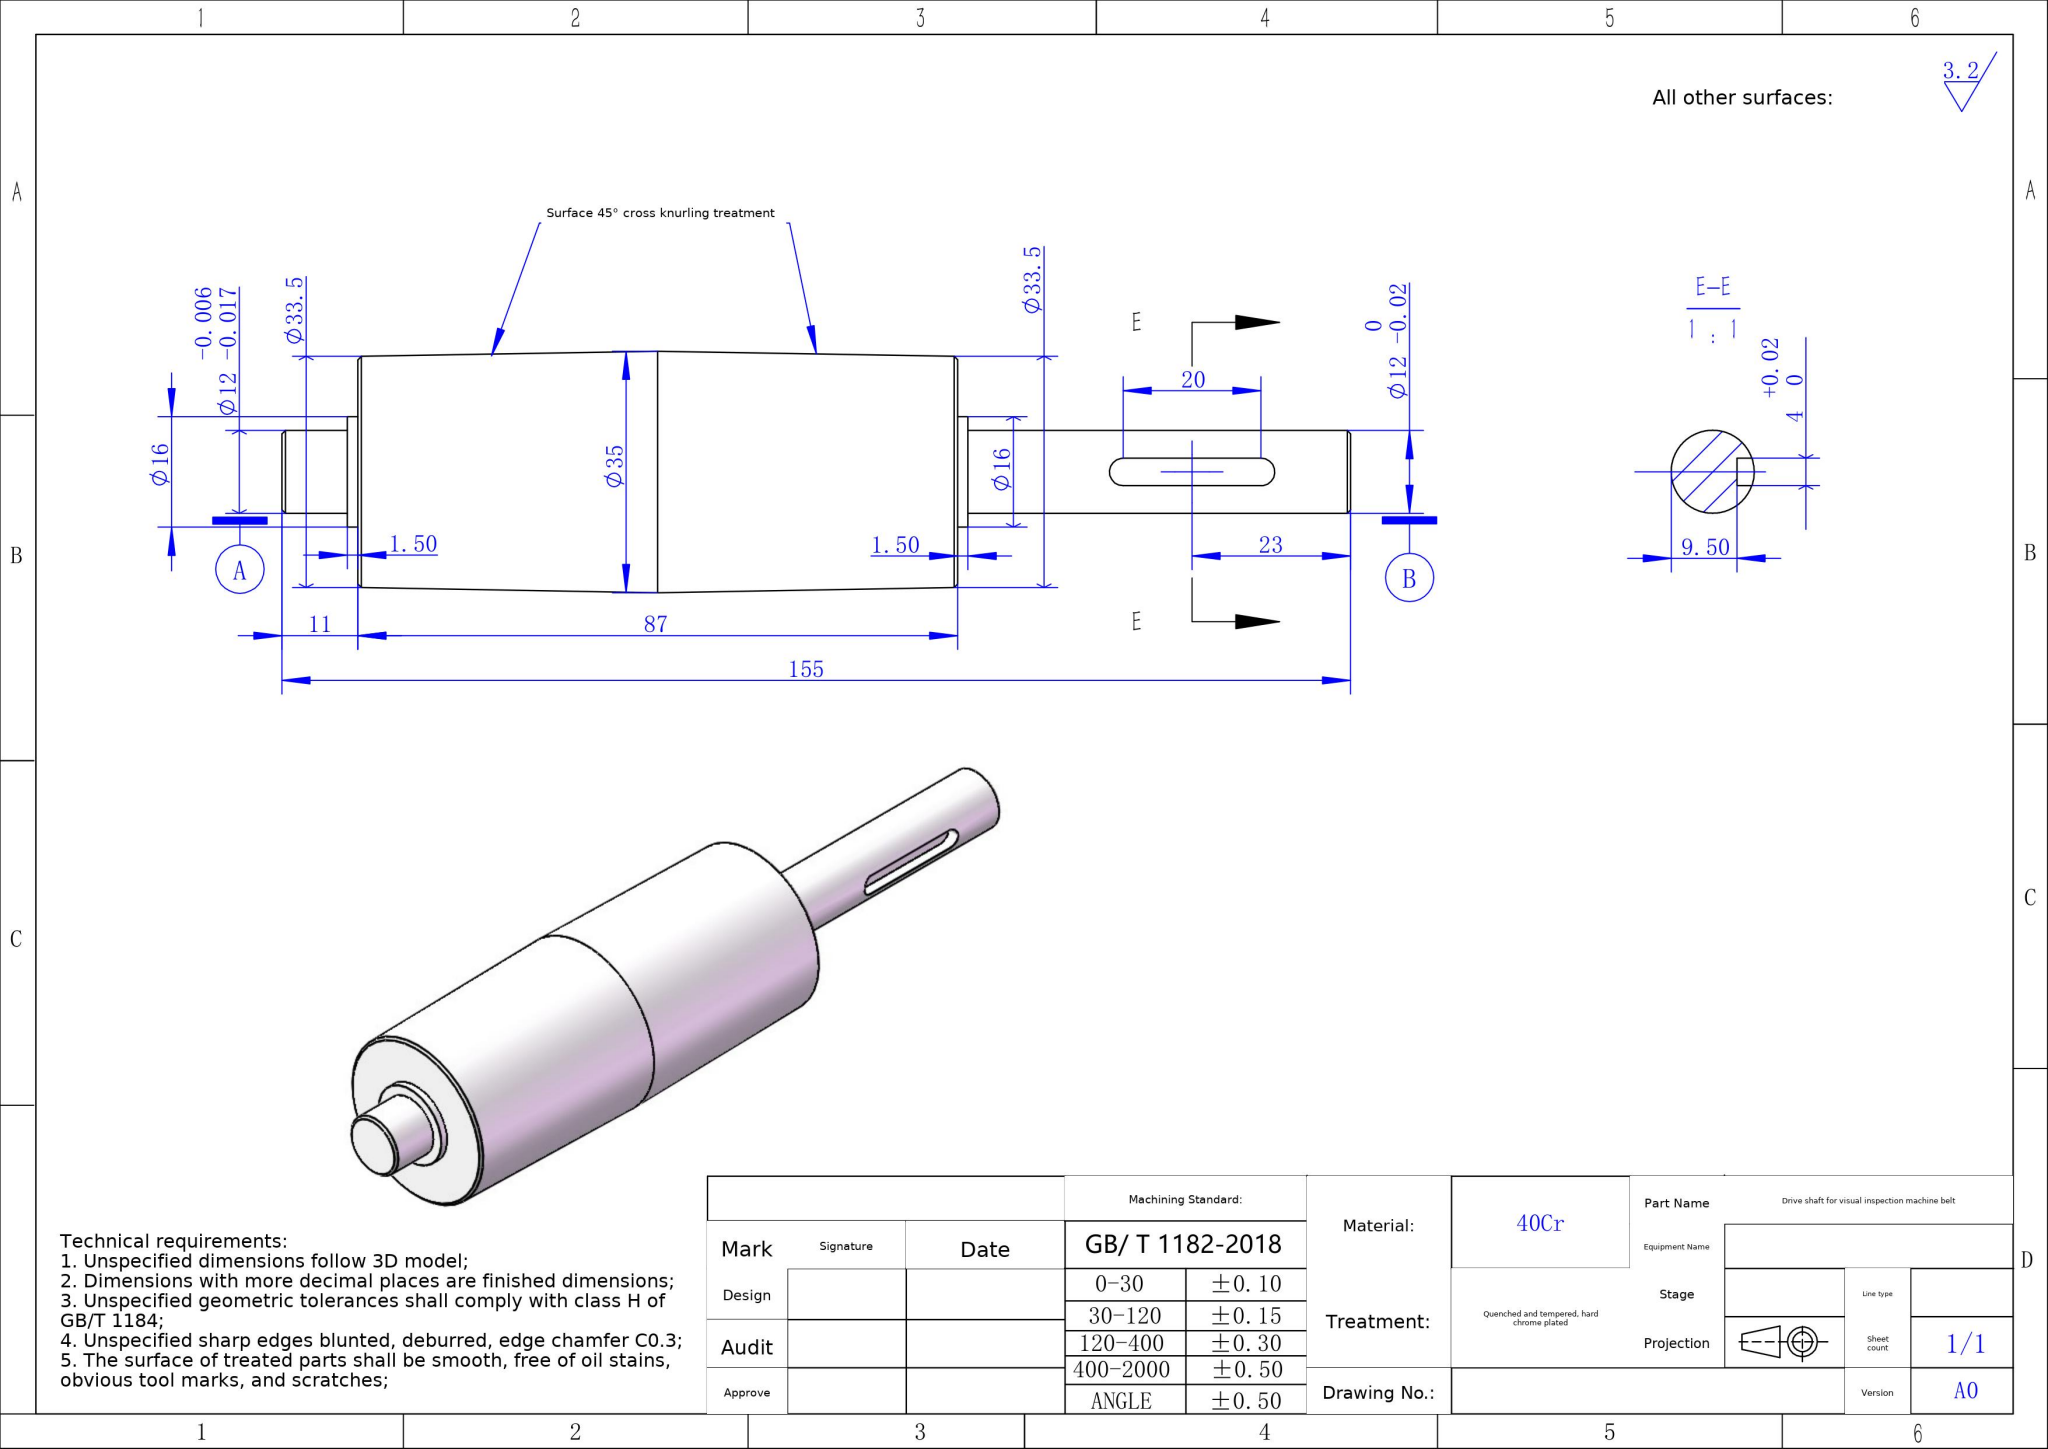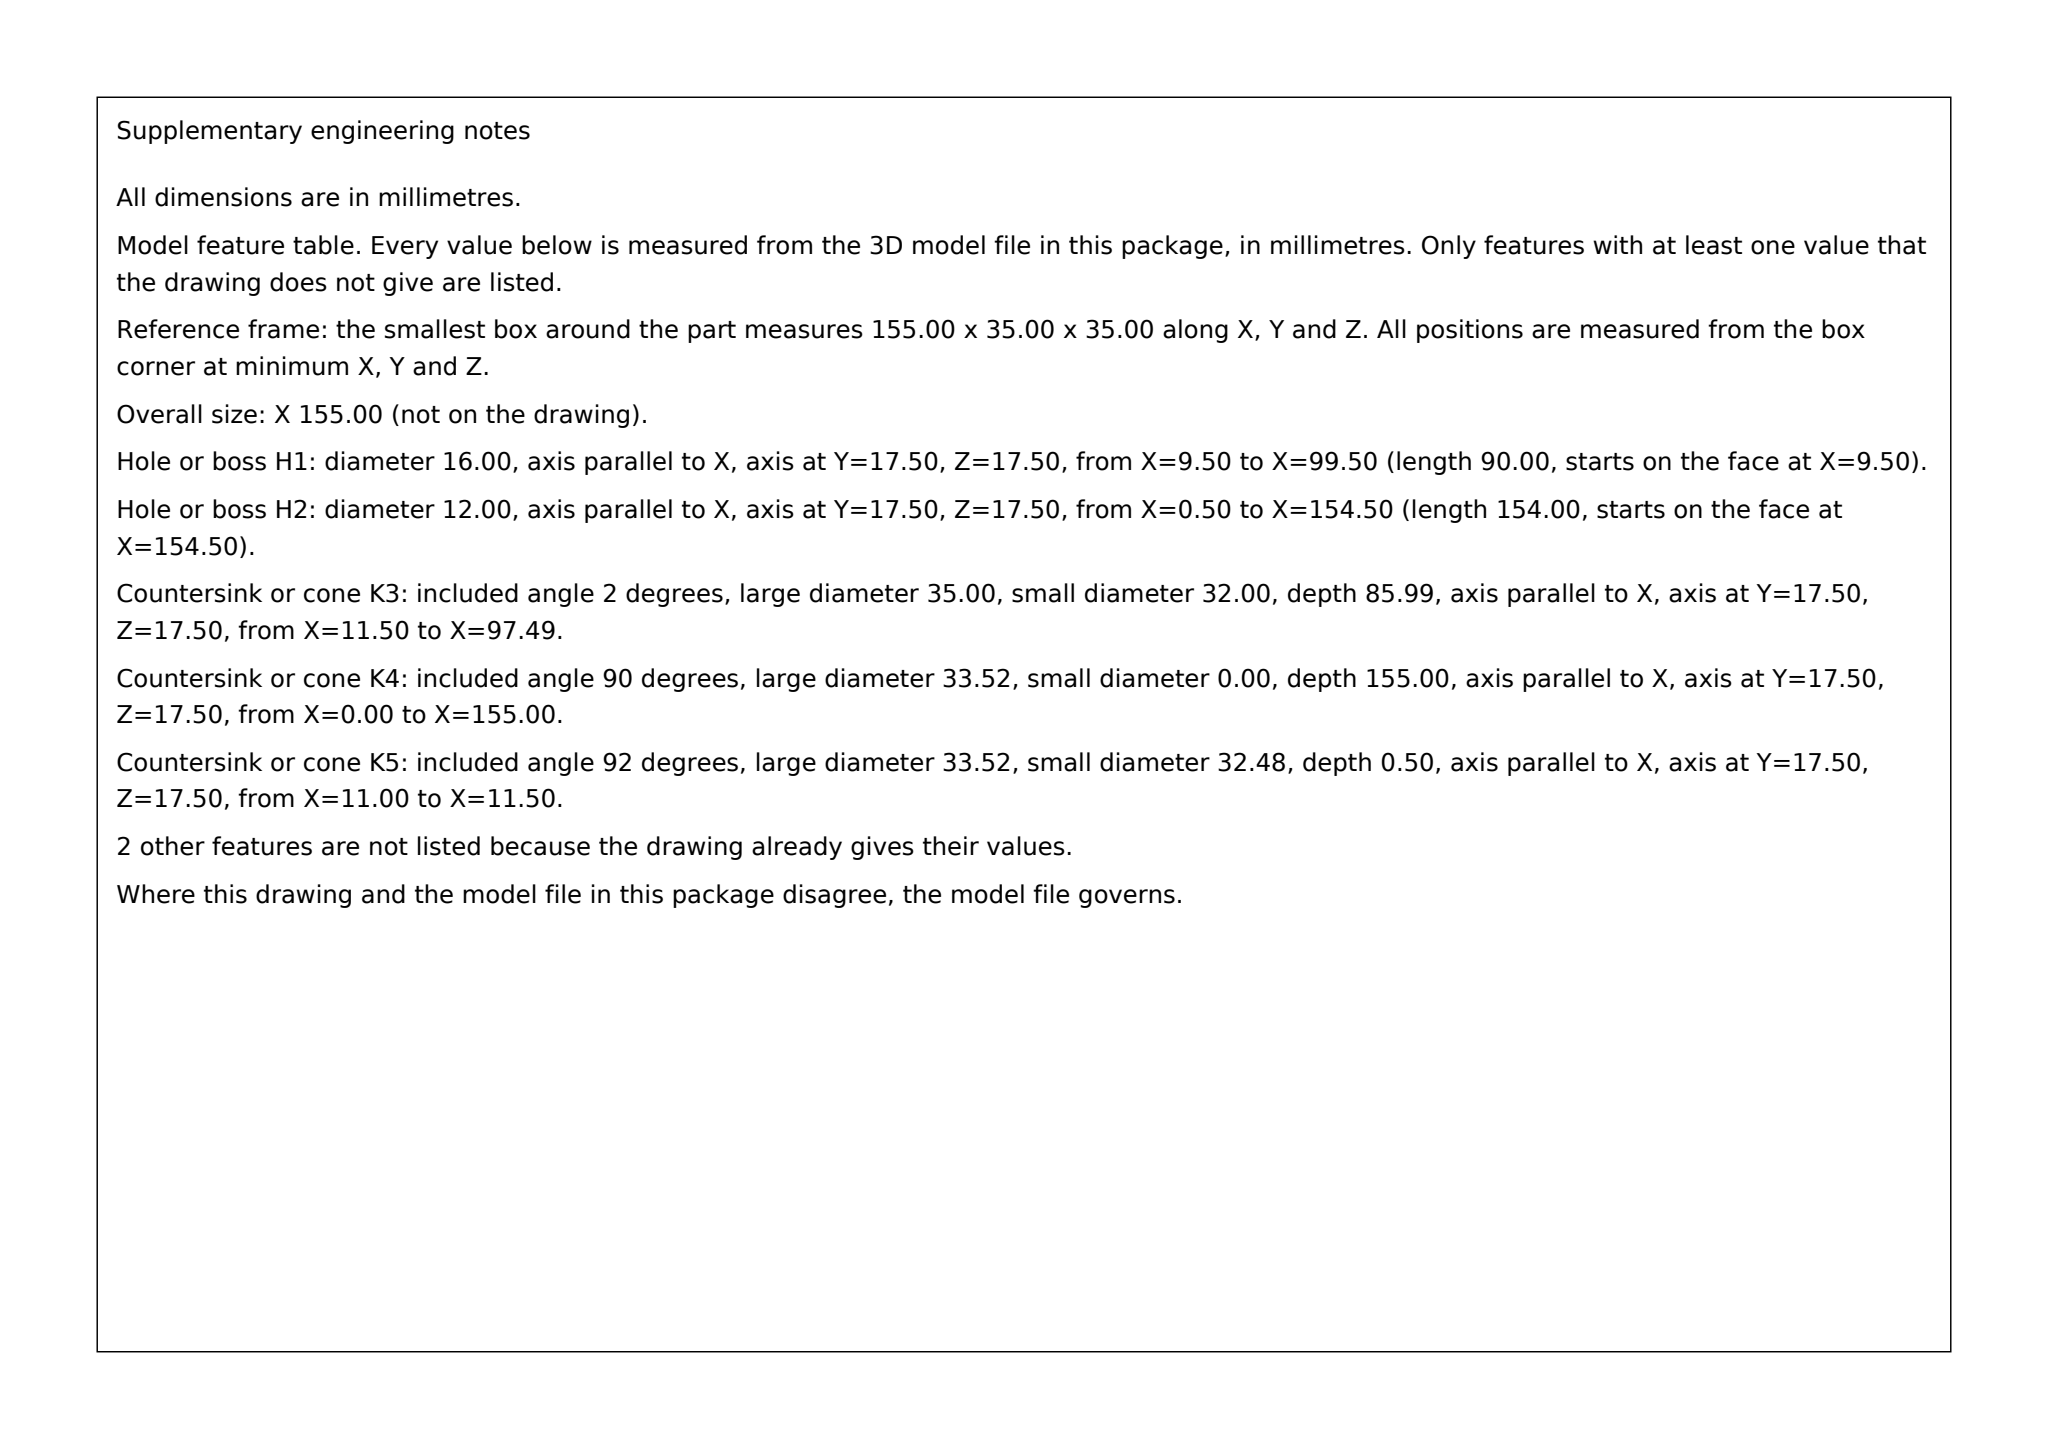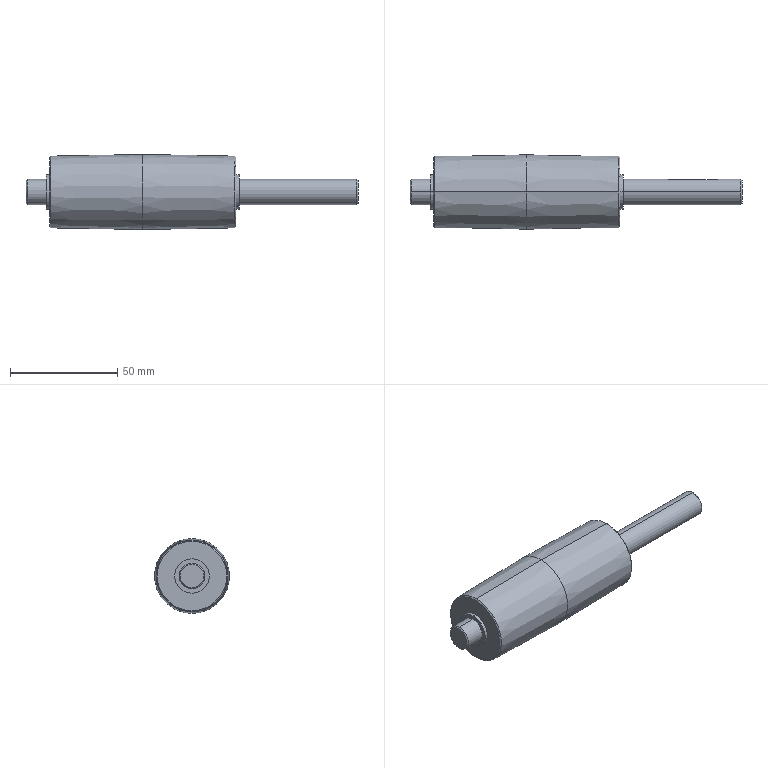Part | SolidWorks | mm | material 40Cr | 1 solid | 31 faces | box 155 x 35 x 35 mm | volume 87865 mm3 | cone 12 | cylinder 10 | plane 9 | commonest cylinder face diameters 12 x4 16 x4 4 x2
build123d program:
from build123d import *
from OCP.BRepFilletAPI import BRepFilletAPI_MakeChamfer

# Parameters (mm, degrees)
CUT_EXTRUDE1_DEPTH = 2.5
CHAMFER1_SIZE      = 0.5
CHAMFER1_SIZE2     = 0.5088


with BuildPart() as part:
    # Sketch1 → Revolve1 (revolve)
    with BuildSketch(Plane.XY, mode=Mode.PRIVATE) as revolve1_sk:
        Polygon((0, 0), (0, 6), (9.5, 6), (9.5, 8), (11, 8), (11, 16.75), (54.5, 17.5), (98, 16.75), (98, 8), (99.5, 8), (99.5, 6), (155, 6), (155, 0), align=None)
    revolve(revolve1_sk.sketch.rotate(Axis((0, 0, 0), (1, 0, 0)), 90), axis=Axis((0, 0, 0), (1, 0, 0)))

    # Sketch3 → Cut-Extrude1 (cut)
    with BuildSketch(Plane(origin=(155, 6, 0), x_dir=(1, 0, 0), z_dir=(0, 1, 0))):
        with BuildLine():
            Line((-33, 2), (-13, 2))
            ThreePointArc((-13, 2), (-11, 0), (-13, -2))
            Line((-13, -2), (-33, -2))
            ThreePointArc((-33, -2), (-35, 0), (-33, 2))
        make_face()
    extrude(amount=-CUT_EXTRUDE1_DEPTH, mode=Mode.SUBTRACT)

    # Chamfer1: one chamfer whose edges measure the first distance from different faces: ONE call of the kernel's chamfer builder (chamfer() names one face for all edges)
    chamfer1_edges_1 = [part.edges().sort_by_distance(p)[0] for p in [
        (155, 0, -6),
        (0, 0, -6),
    ]]
    chamfer1_edges_2 = [part.edges().sort_by_distance(p)[0] for p in [
        (98, 0, -16.75),
    ]]
    chamfer1_side_2 = [part.faces().sort_by_distance(p)[0] for p in [
        (98, 0, -16.276),
    ]]
    chamfer1_edges_3 = [part.edges().sort_by_distance(p)[0] for p in [
        (11, 0, -16.75),
    ]]
    chamfer1_side_3 = [part.faces().sort_by_distance(p)[0] for p in [
        (32.75, 0, -17.125),
    ]]
    chamfer1 = BRepFilletAPI_MakeChamfer(part.part.solid().wrapped)
    for e in chamfer1_edges_1:
        chamfer1.Add(CHAMFER1_SIZE, e.wrapped)
    for e in chamfer1_edges_2:
        chamfer1.Add(CHAMFER1_SIZE, CHAMFER1_SIZE2, e.wrapped, chamfer1_side_2[0].wrapped)  # the first distance lies on this face
    for e in chamfer1_edges_3:
        chamfer1.Add(CHAMFER1_SIZE, CHAMFER1_SIZE2, e.wrapped, chamfer1_side_3[0].wrapped)  # the first distance lies on this face
    add(Compound.cast(chamfer1.Shape()), mode=Mode.REPLACE)


solid = part.part
STEP:
#1=CARTESIAN_POINT('',(0.,0.,5.5));
#2=VERTEX_POINT('',#1);
#3=CARTESIAN_POINT('',(0.,0.,-5.5));
#4=VERTEX_POINT('',#3);
#5=CARTESIAN_POINT('',(0.,0.,0.));
#6=DIRECTION('',(-1.,0.,0.));
#7=DIRECTION('',(0.,0.,-1.));
#8=AXIS2_PLACEMENT_3D('',#5,#6,#7);
#9=CIRCLE('',#8,5.5);
#10=EDGE_CURVE('',#2,#4,#9,.T.);
#11=ORIENTED_EDGE('',*,*,#10,.F.);
#12=CARTESIAN_POINT('',(0.5,0.,6.));
#13=VERTEX_POINT('',#12);
#14=CARTESIAN_POINT('',(0.,0.,5.5));
#15=DIRECTION('',(0.7071,0.,0.7071));
#16=VECTOR('',#15,1000.);
#17=LINE('',#14,#16);
#18=EDGE_CURVE('',#2,#13,#17,.T.);
#19=ORIENTED_EDGE('',*,*,#18,.T.);
#20=CARTESIAN_POINT('',(0.5,0.,-6.));
#21=VERTEX_POINT('',#20);
#22=CARTESIAN_POINT('',(0.5,0.,0.));
#23=DIRECTION('',(1.,0.,0.));
#24=DIRECTION('',(0.,0.,-1.));
#25=AXIS2_PLACEMENT_3D('',#22,#23,#24);
#26=CIRCLE('',#25,6.);
#27=EDGE_CURVE('',#21,#13,#26,.T.);
#28=ORIENTED_EDGE('',*,*,#27,.F.);
#29=CARTESIAN_POINT('',(0.,0.,-5.5));
#30=DIRECTION('',(0.7071,0.,-0.7071));
#31=VECTOR('',#30,1000.);
#32=LINE('',#29,#31);
#33=EDGE_CURVE('',#4,#21,#32,.T.);
#34=ORIENTED_EDGE('',*,*,#33,.F.);
#35=EDGE_LOOP('',(#11,#19,#28,#34));
#36=FACE_OUTER_BOUND('',#35,.T.);
#37=CARTESIAN_POINT('',(0.,0.,0.));
#38=DIRECTION('',(1.,0.,0.));
#39=DIRECTION('',(0.,0.,-1.));
#40=AXIS2_PLACEMENT_3D('',#37,#38,#39);
#41=CONICAL_SURFACE('',#40,5.5,0.7854);
#42=ADVANCED_FACE('',(#36),#41,.T.);
#43=CARTESIAN_POINT('',(155.,0.,-5.5));
#44=VERTEX_POINT('',#43);
#45=CARTESIAN_POINT('',(155.,0.,5.5));
#46=VERTEX_POINT('',#45);
#47=CARTESIAN_POINT('',(155.,0.,0.));
#48=DIRECTION('',(1.,0.,0.));
#49=DIRECTION('',(0.,0.,1.));
#50=AXIS2_PLACEMENT_3D('',#47,#48,#49);
#51=CIRCLE('',#50,5.5);
#52=EDGE_CURVE('',#44,#46,#51,.T.);
#53=ORIENTED_EDGE('',*,*,#52,.F.);
#54=CARTESIAN_POINT('',(154.5,0.,-6.));
#55=VERTEX_POINT('',#54);
#56=CARTESIAN_POINT('',(154.5,0.,-6.));
#57=DIRECTION('',(-0.7071,0.,-0.7071));
#58=VECTOR('',#57,1000.);
#59=LINE('',#56,#58);
#60=EDGE_CURVE('',#44,#55,#59,.T.);
#61=ORIENTED_EDGE('',*,*,#60,.T.);
#62=CARTESIAN_POINT('',(154.5,0.,6.));
#63=VERTEX_POINT('',#62);
#64=CARTESIAN_POINT('',(154.5,0.,0.));
#65=DIRECTION('',(-1.,0.,0.));
#66=DIRECTION('',(0.,0.,1.));
#67=AXIS2_PLACEMENT_3D('',#64,#65,#66);
#68=CIRCLE('',#67,6.);
#69=EDGE_CURVE('',#63,#55,#68,.T.);
#70=ORIENTED_EDGE('',*,*,#69,.F.);
#71=CARTESIAN_POINT('',(154.5,0.,6.));
#72=DIRECTION('',(-0.7071,0.,0.7071));
#73=VECTOR('',#72,1000.);
#74=LINE('',#71,#73);
#75=EDGE_CURVE('',#46,#63,#74,.T.);
#76=ORIENTED_EDGE('',*,*,#75,.F.);
#77=EDGE_LOOP('',(#53,#61,#70,#76));
#78=FACE_OUTER_BOUND('',#77,.T.);
#79=CARTESIAN_POINT('',(154.5,0.,0.));
#80=DIRECTION('',(-1.,0.,0.));
#81=DIRECTION('',(0.,0.,1.));
#82=AXIS2_PLACEMENT_3D('',#79,#80,#81);
#83=CONICAL_SURFACE('',#82,6.,0.7854);
#84=ADVANCED_FACE('',(#78),#83,.T.);
#85=CARTESIAN_POINT('',(98.,0.,-16.25));
#86=VERTEX_POINT('',#85);
#87=CARTESIAN_POINT('',(98.,0.,16.25));
#88=VERTEX_POINT('',#87);
#89=CARTESIAN_POINT('',(98.,0.,0.));
#90=DIRECTION('',(1.,0.,0.));
#91=DIRECTION('',(0.,0.,1.));
#92=AXIS2_PLACEMENT_3D('',#89,#90,#91);
#93=CIRCLE('',#92,16.25);
#94=EDGE_CURVE('',#86,#88,#93,.T.);
#95=ORIENTED_EDGE('',*,*,#94,.F.);
#96=CARTESIAN_POINT('',(97.491,0.,-16.759));
#97=VERTEX_POINT('',#96);
#98=CARTESIAN_POINT('',(97.491,0.,-16.759));
#99=DIRECTION('',(-0.7071,0.,-0.7071));
#100=VECTOR('',#99,1000.);
#101=LINE('',#98,#100);
#102=EDGE_CURVE('',#86,#97,#101,.T.);
#103=ORIENTED_EDGE('',*,*,#102,.T.);
#104=CARTESIAN_POINT('',(97.491,0.,16.759));
#105=VERTEX_POINT('',#104);
#106=CARTESIAN_POINT('',(97.491,0.,0.));
#107=DIRECTION('',(-1.,0.,0.));
#108=DIRECTION('',(0.,0.,-1.));
#109=AXIS2_PLACEMENT_3D('',#106,#107,#108);
#110=CIRCLE('',#109,16.759);
#111=EDGE_CURVE('',#105,#97,#110,.T.);
#112=ORIENTED_EDGE('',*,*,#111,.F.);
#113=CARTESIAN_POINT('',(97.491,0.,16.759));
#114=DIRECTION('',(-0.7071,0.,0.7071));
#115=VECTOR('',#114,1000.);
#116=LINE('',#113,#115);
#117=EDGE_CURVE('',#88,#105,#116,.T.);
#118=ORIENTED_EDGE('',*,*,#117,.F.);
#119=EDGE_LOOP('',(#95,#103,#112,#118));
#120=FACE_OUTER_BOUND('',#119,.T.);
#121=CARTESIAN_POINT('',(97.491,0.,0.));
#122=DIRECTION('',(-1.,0.,0.));
#123=DIRECTION('',(0.,0.,1.));
#124=AXIS2_PLACEMENT_3D('',#121,#122,#123);
#125=CONICAL_SURFACE('',#124,16.759,0.7854);
#126=ADVANCED_FACE('',(#120),#125,.T.);
#127=CARTESIAN_POINT('',(11.,0.,16.241));
#128=VERTEX_POINT('',#127);
#129=CARTESIAN_POINT('',(11.,0.,-16.241));
#130=VERTEX_POINT('',#129);
#131=CARTESIAN_POINT('',(11.,0.,0.));
#132=DIRECTION('',(-1.,0.,0.));
#133=DIRECTION('',(0.,0.,-1.));
#134=AXIS2_PLACEMENT_3D('',#131,#132,#133);
#135=CIRCLE('',#134,16.241);
#136=EDGE_CURVE('',#128,#130,#135,.T.);
#137=ORIENTED_EDGE('',*,*,#136,.F.);
#138=CARTESIAN_POINT('',(11.5,0.,16.759));
#139=VERTEX_POINT('',#138);
#140=CARTESIAN_POINT('',(11.,0.,16.241));
#141=DIRECTION('',(0.6948,0.,0.7192));
#142=VECTOR('',#141,1000.);
#143=LINE('',#140,#142);
#144=EDGE_CURVE('',#128,#139,#143,.T.);
#145=ORIENTED_EDGE('',*,*,#144,.T.);
#146=CARTESIAN_POINT('',(11.5,0.,-16.759));
#147=VERTEX_POINT('',#146);
#148=CARTESIAN_POINT('',(11.5,0.,0.));
#149=DIRECTION('',(1.,0.,0.));
#150=DIRECTION('',(0.,0.,1.));
#151=AXIS2_PLACEMENT_3D('',#148,#149,#150);
#152=CIRCLE('',#151,16.759);
#153=EDGE_CURVE('',#147,#139,#152,.T.);
#154=ORIENTED_EDGE('',*,*,#153,.F.);
#155=CARTESIAN_POINT('',(11.,0.,-16.241));
#156=DIRECTION('',(0.6948,0.,-0.7192));
#157=VECTOR('',#156,1000.);
#158=LINE('',#155,#157);
#159=EDGE_CURVE('',#130,#147,#158,.T.);
#160=ORIENTED_EDGE('',*,*,#159,.F.);
#161=EDGE_LOOP('',(#137,#145,#154,#160));
#162=FACE_OUTER_BOUND('',#161,.T.);
#163=CARTESIAN_POINT('',(11.,0.,0.));
#164=DIRECTION('',(1.,0.,0.));
#165=DIRECTION('',(0.,0.,-1.));
#166=AXIS2_PLACEMENT_3D('',#163,#164,#165);
#167=CONICAL_SURFACE('',#166,16.241,0.8026);
#168=ADVANCED_FACE('',(#162),#167,.T.);
#169=CARTESIAN_POINT('',(122.,5.657,-2.));
#170=VERTEX_POINT('',#169);
#171=CARTESIAN_POINT('',(142.,5.657,-2.));
#172=VERTEX_POINT('',#171);
#173=CARTESIAN_POINT('',(0.,5.657,-2.));
#174=DIRECTION('',(1.,0.,0.));
#175=VECTOR('',#174,1000.);
#176=LINE('',#173,#175);
#177=EDGE_CURVE('',#170,#172,#176,.T.);
#178=ORIENTED_EDGE('',*,*,#177,.T.);
#179=CARTESIAN_POINT('',(142.,5.657,2.));
#180=VERTEX_POINT('',#179);
#181=CARTESIAN_POINT('',(142.,5.657,-2.));
#182=CARTESIAN_POINT('',(142.133,5.657,-2.));
#183=CARTESIAN_POINT('',(142.264,5.662,-1.987));
#184=CARTESIAN_POINT('',(142.521,5.679,-1.935));
#185=CARTESIAN_POINT('',(142.648,5.693,-1.897));
#186=CARTESIAN_POINT('',(142.89,5.725,-1.796));
#187=CARTESIAN_POINT('',(143.004,5.744,-1.735));
#188=CARTESIAN_POINT('',(143.221,5.786,-1.59));
#189=CARTESIAN_POINT('',(143.323,5.809,-1.506));
#190=CARTESIAN_POINT('',(143.597,5.875,-1.231));
#191=CARTESIAN_POINT('',(143.746,5.919,-1.01));
#192=CARTESIAN_POINT('',(143.896,5.966,-0.6496));
#193=CARTESIAN_POINT('',(143.935,5.979,-0.5226));
#194=CARTESIAN_POINT('',(143.987,5.996,-0.264));
#195=CARTESIAN_POINT('',(144.,6.,-0.1336));
#196=CARTESIAN_POINT('',(144.,6.,0.1294));
#197=CARTESIAN_POINT('',(143.987,5.996,0.2629));
#198=CARTESIAN_POINT('',(143.936,5.979,0.5202));
#199=CARTESIAN_POINT('',(143.898,5.966,0.6454));
#200=CARTESIAN_POINT('',(143.796,5.935,0.8889));
#201=CARTESIAN_POINT('',(143.734,5.916,1.004));
#202=CARTESIAN_POINT('',(143.59,5.876,1.22));
#203=CARTESIAN_POINT('',(143.507,5.853,1.322));
#204=CARTESIAN_POINT('',(143.323,5.809,1.506));
#205=CARTESIAN_POINT('',(143.223,5.787,1.588));
#206=CARTESIAN_POINT('',(143.007,5.745,1.733));
#207=CARTESIAN_POINT('',(142.89,5.725,1.796));
#208=CARTESIAN_POINT('',(142.529,5.677,1.946));
#209=CARTESIAN_POINT('',(142.266,5.657,2.));
#210=CARTESIAN_POINT('',(142.,5.657,2.));
#211=B_SPLINE_CURVE_WITH_KNOTS('',3,(#181,#182,#183,#184,#185,#186,#187,#188,#189,#190,#191,#192,#193,#194,#195,#196,#197,#198,#199,#200,#201,#202,#203,#204,#205,#206,#207,#208,#209,#210),.UNSPECIFIED.,.F.,.F.,(4,2,2,2,2,2,2,2,2,2,2,2,2,2,4),(0.,0.0003935,0.000787,0.00118,0.001574,0.002361,0.002754,0.003148,0.003541,0.003935,0.004328,0.004722,0.005115,0.005509,0.006296),.UNSPECIFIED.);
#212=EDGE_CURVE('',#172,#180,#211,.T.);
#213=ORIENTED_EDGE('',*,*,#212,.T.);
#214=CARTESIAN_POINT('',(122.,5.657,2.));
#215=VERTEX_POINT('',#214);
#216=CARTESIAN_POINT('',(0.,5.657,2.));
#217=DIRECTION('',(-1.,0.,0.));
#218=VECTOR('',#217,1000.);
#219=LINE('',#216,#218);
#220=EDGE_CURVE('',#180,#215,#219,.T.);
#221=ORIENTED_EDGE('',*,*,#220,.T.);
#222=CARTESIAN_POINT('',(122.,5.657,2.));
#223=CARTESIAN_POINT('',(121.867,5.657,2.));
#224=CARTESIAN_POINT('',(121.736,5.662,1.987));
#225=CARTESIAN_POINT('',(121.479,5.679,1.935));
#226=CARTESIAN_POINT('',(121.352,5.693,1.897));
#227=CARTESIAN_POINT('',(121.11,5.725,1.796));
#228=CARTESIAN_POINT('',(120.996,5.744,1.735));
#229=CARTESIAN_POINT('',(120.779,5.786,1.59));
#230=CARTESIAN_POINT('',(120.677,5.809,1.506));
#231=CARTESIAN_POINT('',(120.403,5.875,1.231));
#232=CARTESIAN_POINT('',(120.254,5.919,1.01));
#233=CARTESIAN_POINT('',(120.104,5.966,0.6496));
#234=CARTESIAN_POINT('',(120.065,5.979,0.5226));
#235=CARTESIAN_POINT('',(120.013,5.996,0.264));
#236=CARTESIAN_POINT('',(120.,6.,0.1336));
#237=CARTESIAN_POINT('',(120.,6.,-0.1294));
#238=CARTESIAN_POINT('',(120.013,5.996,-0.2629));
#239=CARTESIAN_POINT('',(120.064,5.979,-0.5202));
#240=CARTESIAN_POINT('',(120.102,5.966,-0.6454));
#241=CARTESIAN_POINT('',(120.204,5.935,-0.8889));
#242=CARTESIAN_POINT('',(120.266,5.916,-1.004));
#243=CARTESIAN_POINT('',(120.41,5.876,-1.22));
#244=CARTESIAN_POINT('',(120.493,5.853,-1.322));
#245=CARTESIAN_POINT('',(120.677,5.809,-1.506));
#246=CARTESIAN_POINT('',(120.777,5.787,-1.588));
#247=CARTESIAN_POINT('',(120.993,5.745,-1.733));
#248=CARTESIAN_POINT('',(121.11,5.725,-1.796));
#249=CARTESIAN_POINT('',(121.471,5.677,-1.946));
#250=CARTESIAN_POINT('',(121.734,5.657,-2.));
#251=CARTESIAN_POINT('',(122.,5.657,-2.));
#252=B_SPLINE_CURVE_WITH_KNOTS('',3,(#222,#223,#224,#225,#226,#227,#228,#229,#230,#231,#232,#233,#234,#235,#236,#237,#238,#239,#240,#241,#242,#243,#244,#245,#246,#247,#248,#249,#250,#251),.UNSPECIFIED.,.F.,.F.,(4,2,2,2,2,2,2,2,2,2,2,2,2,2,4),(0.,0.0003935,0.000787,0.00118,0.001574,0.002361,0.002754,0.003148,0.003541,0.003935,0.004328,0.004722,0.005115,0.005509,0.006296),.UNSPECIFIED.);
#253=EDGE_CURVE('',#215,#170,#252,.T.);
#254=ORIENTED_EDGE('',*,*,#253,.T.);
#255=EDGE_LOOP('',(#178,#213,#221,#254));
#256=FACE_BOUND('',#255,.T.);
#257=ORIENTED_EDGE('',*,*,#69,.T.);
#258=CARTESIAN_POINT('',(99.5,0.,-6.));
#259=VERTEX_POINT('',#258);
#260=CARTESIAN_POINT('',(0.,0.,-6.));
#261=DIRECTION('',(-1.,0.,0.));
#262=VECTOR('',#261,1000.);
#263=LINE('',#260,#262);
#264=EDGE_CURVE('',#55,#259,#263,.T.);
#265=ORIENTED_EDGE('',*,*,#264,.T.);
#266=CARTESIAN_POINT('',(99.5,0.,6.));
#267=VERTEX_POINT('',#266);
#268=CARTESIAN_POINT('',(99.5,0.,0.));
#269=DIRECTION('',(-1.,0.,0.));
#270=DIRECTION('',(0.,0.,1.));
#271=AXIS2_PLACEMENT_3D('',#268,#269,#270);
#272=CIRCLE('',#271,6.);
#273=EDGE_CURVE('',#267,#259,#272,.T.);
#274=ORIENTED_EDGE('',*,*,#273,.F.);
#275=CARTESIAN_POINT('',(0.,0.,6.));
#276=DIRECTION('',(-1.,0.,0.));
#277=VECTOR('',#276,1000.);
#278=LINE('',#275,#277);
#279=EDGE_CURVE('',#63,#267,#278,.T.);
#280=ORIENTED_EDGE('',*,*,#279,.F.);
#281=EDGE_LOOP('',(#257,#265,#274,#280));
#282=FACE_OUTER_BOUND('',#281,.T.);
#283=CARTESIAN_POINT('',(0.,0.,0.));
#284=DIRECTION('',(-1.,0.,0.));
#285=DIRECTION('',(0.,0.,1.));
#286=AXIS2_PLACEMENT_3D('',#283,#284,#285);
#287=CYLINDRICAL_SURFACE('',#286,6.);
#288=ADVANCED_FACE('',(#256,#282),#287,.T.);
#289=CARTESIAN_POINT('',(99.5,0.,8.));
#290=VERTEX_POINT('',#289);
#291=CARTESIAN_POINT('',(99.5,0.,-8.));
#292=VERTEX_POINT('',#291);
#293=CARTESIAN_POINT('',(99.5,0.,0.));
#294=DIRECTION('',(-1.,0.,0.));
#295=DIRECTION('',(0.,0.,1.));
#296=AXIS2_PLACEMENT_3D('',#293,#294,#295);
#297=CIRCLE('',#296,8.);
#298=EDGE_CURVE('',#290,#292,#297,.T.);
#299=ORIENTED_EDGE('',*,*,#298,.T.);
#300=CARTESIAN_POINT('',(98.,0.,-8.));
#301=VERTEX_POINT('',#300);
#302=CARTESIAN_POINT('',(0.,0.,-8.));
#303=DIRECTION('',(-1.,0.,0.));
#304=VECTOR('',#303,1000.);
#305=LINE('',#302,#304);
#306=EDGE_CURVE('',#292,#301,#305,.T.);
#307=ORIENTED_EDGE('',*,*,#306,.T.);
#308=CARTESIAN_POINT('',(98.,0.,8.));
#309=VERTEX_POINT('',#308);
#310=CARTESIAN_POINT('',(98.,0.,0.));
#311=DIRECTION('',(-1.,0.,0.));
#312=DIRECTION('',(0.,0.,1.));
#313=AXIS2_PLACEMENT_3D('',#310,#311,#312);
#314=CIRCLE('',#313,8.);
#315=EDGE_CURVE('',#309,#301,#314,.T.);
#316=ORIENTED_EDGE('',*,*,#315,.F.);
#317=CARTESIAN_POINT('',(0.,0.,8.));
#318=DIRECTION('',(-1.,0.,0.));
#319=VECTOR('',#318,1000.);
#320=LINE('',#317,#319);
#321=EDGE_CURVE('',#290,#309,#320,.T.);
#322=ORIENTED_EDGE('',*,*,#321,.F.);
#323=EDGE_LOOP('',(#299,#307,#316,#322));
#324=FACE_OUTER_BOUND('',#323,.T.);
#325=CARTESIAN_POINT('',(0.,0.,0.));
#326=DIRECTION('',(-1.,0.,0.));
#327=DIRECTION('',(0.,0.,1.));
#328=AXIS2_PLACEMENT_3D('',#325,#326,#327);
#329=CYLINDRICAL_SURFACE('',#328,8.);
#330=ADVANCED_FACE('',(#324),#329,.T.);
#331=ORIENTED_EDGE('',*,*,#111,.T.);
#332=CARTESIAN_POINT('',(54.5,0.,-17.5));
#333=VERTEX_POINT('',#332);
#334=CARTESIAN_POINT('',(98.,0.,-16.75));
#335=DIRECTION('',(-0.9999,0.,-0.01724));
#336=VECTOR('',#335,1000.);
#337=LINE('',#334,#336);
#338=EDGE_CURVE('',#97,#333,#337,.T.);
#339=ORIENTED_EDGE('',*,*,#338,.T.);
#340=CARTESIAN_POINT('',(54.5,0.,17.5));
#341=VERTEX_POINT('',#340);
#342=CARTESIAN_POINT('',(54.5,0.,0.));
#343=DIRECTION('',(-1.,0.,0.));
#344=DIRECTION('',(0.,0.,1.));
#345=AXIS2_PLACEMENT_3D('',#342,#343,#344);
#346=CIRCLE('',#345,17.5);
#347=EDGE_CURVE('',#341,#333,#346,.T.);
#348=ORIENTED_EDGE('',*,*,#347,.F.);
#349=CARTESIAN_POINT('',(98.,0.,16.75));
#350=DIRECTION('',(-0.9999,0.,0.01724));
#351=VECTOR('',#350,1000.);
#352=LINE('',#349,#351);
#353=EDGE_CURVE('',#105,#341,#352,.T.);
#354=ORIENTED_EDGE('',*,*,#353,.F.);
#355=EDGE_LOOP('',(#331,#339,#348,#354));
#356=FACE_OUTER_BOUND('',#355,.T.);
#357=CARTESIAN_POINT('',(98.,0.,0.));
#358=DIRECTION('',(-1.,0.,0.));
#359=DIRECTION('',(0.,0.,1.));
#360=AXIS2_PLACEMENT_3D('',#357,#358,#359);
#361=CONICAL_SURFACE('',#360,16.75,0.01724);
#362=ADVANCED_FACE('',(#356),#361,.T.);
#363=ORIENTED_EDGE('',*,*,#153,.T.);
#364=CARTESIAN_POINT('',(54.5,0.,17.5));
#365=DIRECTION('',(0.9999,0.,0.01724));
#366=VECTOR('',#365,1000.);
#367=LINE('',#364,#366);
#368=EDGE_CURVE('',#139,#341,#367,.T.);
#369=ORIENTED_EDGE('',*,*,#368,.T.);
#370=ORIENTED_EDGE('',*,*,#347,.T.);
#371=CARTESIAN_POINT('',(54.5,0.,-17.5));
#372=DIRECTION('',(0.9999,0.,-0.01724));
#373=VECTOR('',#372,1000.);
#374=LINE('',#371,#373);
#375=EDGE_CURVE('',#147,#333,#374,.T.);
#376=ORIENTED_EDGE('',*,*,#375,.F.);
#377=EDGE_LOOP('',(#363,#369,#370,#376));
#378=FACE_OUTER_BOUND('',#377,.T.);
#379=CARTESIAN_POINT('',(54.5,0.,0.));
#380=DIRECTION('',(1.,0.,0.));
#381=DIRECTION('',(0.,0.,-1.));
#382=AXIS2_PLACEMENT_3D('',#379,#380,#381);
#383=CONICAL_SURFACE('',#382,17.5,0.01724);
#384=ADVANCED_FACE('',(#378),#383,.T.);
#385=CARTESIAN_POINT('',(11.,0.,8.));
#386=VERTEX_POINT('',#385);
#387=CARTESIAN_POINT('',(11.,0.,-8.));
#388=VERTEX_POINT('',#387);
#389=CARTESIAN_POINT('',(11.,0.,0.));
#390=DIRECTION('',(-1.,0.,0.));
#391=DIRECTION('',(0.,0.,1.));
#392=AXIS2_PLACEMENT_3D('',#389,#390,#391);
#393=CIRCLE('',#392,8.);
#394=EDGE_CURVE('',#386,#388,#393,.T.);
#395=ORIENTED_EDGE('',*,*,#394,.T.);
#396=CARTESIAN_POINT('',(9.5,0.,-8.));
#397=VERTEX_POINT('',#396);
#398=CARTESIAN_POINT('',(0.,0.,-8.));
#399=DIRECTION('',(-1.,0.,0.));
#400=VECTOR('',#399,1000.);
#401=LINE('',#398,#400);
#402=EDGE_CURVE('',#388,#397,#401,.T.);
#403=ORIENTED_EDGE('',*,*,#402,.T.);
#404=CARTESIAN_POINT('',(9.5,0.,8.));
#405=VERTEX_POINT('',#404);
#406=CARTESIAN_POINT('',(9.5,0.,0.));
#407=DIRECTION('',(-1.,0.,0.));
#408=DIRECTION('',(0.,0.,1.));
#409=AXIS2_PLACEMENT_3D('',#406,#407,#408);
#410=CIRCLE('',#409,8.);
#411=EDGE_CURVE('',#405,#397,#410,.T.);
#412=ORIENTED_EDGE('',*,*,#411,.F.);
#413=CARTESIAN_POINT('',(0.,0.,8.));
#414=DIRECTION('',(-1.,0.,0.));
#415=VECTOR('',#414,1000.);
#416=LINE('',#413,#415);
#417=EDGE_CURVE('',#386,#405,#416,.T.);
#418=ORIENTED_EDGE('',*,*,#417,.F.);
#419=EDGE_LOOP('',(#395,#403,#412,#418));
#420=FACE_OUTER_BOUND('',#419,.T.);
#421=CARTESIAN_POINT('',(0.,0.,0.));
#422=DIRECTION('',(-1.,0.,0.));
#423=DIRECTION('',(0.,0.,1.));
#424=AXIS2_PLACEMENT_3D('',#421,#422,#423);
#425=CYLINDRICAL_SURFACE('',#424,8.);
#426=ADVANCED_FACE('',(#420),#425,.T.);
#427=CARTESIAN_POINT('',(9.5,0.,6.));
#428=VERTEX_POINT('',#427);
#429=CARTESIAN_POINT('',(9.5,0.,-6.));
#430=VERTEX_POINT('',#429);
#431=CARTESIAN_POINT('',(9.5,0.,0.));
#432=DIRECTION('',(-1.,0.,0.));
#433=DIRECTION('',(0.,0.,1.));
#434=AXIS2_PLACEMENT_3D('',#431,#432,#433);
#435=CIRCLE('',#434,6.);
#436=EDGE_CURVE('',#428,#430,#435,.T.);
#437=ORIENTED_EDGE('',*,*,#436,.T.);
#438=CARTESIAN_POINT('',(0.,0.,-6.));
#439=DIRECTION('',(-1.,0.,0.));
#440=VECTOR('',#439,1000.);
#441=LINE('',#438,#440);
#442=EDGE_CURVE('',#430,#21,#441,.T.);
#443=ORIENTED_EDGE('',*,*,#442,.T.);
#444=ORIENTED_EDGE('',*,*,#27,.T.);
#445=CARTESIAN_POINT('',(0.,0.,6.));
#446=DIRECTION('',(-1.,0.,0.));
#447=VECTOR('',#446,1000.);
#448=LINE('',#445,#447);
#449=EDGE_CURVE('',#428,#13,#448,.T.);
#450=ORIENTED_EDGE('',*,*,#449,.F.);
#451=EDGE_LOOP('',(#437,#443,#444,#450));
#452=FACE_OUTER_BOUND('',#451,.T.);
#453=CARTESIAN_POINT('',(0.,0.,0.));
#454=DIRECTION('',(-1.,0.,0.));
#455=DIRECTION('',(0.,0.,1.));
#456=AXIS2_PLACEMENT_3D('',#453,#454,#455);
#457=CYLINDRICAL_SURFACE('',#456,6.);
#458=ADVANCED_FACE('',(#452),#457,.T.);
#459=CARTESIAN_POINT('',(0.,0.,0.));
#460=DIRECTION('',(-1.,0.,0.));
#461=DIRECTION('',(0.,0.,-1.));
#462=AXIS2_PLACEMENT_3D('',#459,#460,#461);
#463=CIRCLE('',#462,5.5);
#464=EDGE_CURVE('',#4,#2,#463,.T.);
#465=ORIENTED_EDGE('',*,*,#464,.T.);
#466=ORIENTED_EDGE('',*,*,#10,.T.);
#467=EDGE_LOOP('',(#465,#466));
#468=FACE_OUTER_BOUND('',#467,.T.);
#469=CARTESIAN_POINT('',(0.,0.,0.));
#470=DIRECTION('',(1.,0.,0.));
#471=DIRECTION('',(0.,0.,-1.));
#472=AXIS2_PLACEMENT_3D('',#469,#470,#471);
#473=PLANE('',#472);
#474=ADVANCED_FACE('',(#468),#473,.F.);
#475=ORIENTED_EDGE('',*,*,#442,.F.);
#476=CARTESIAN_POINT('',(9.5,0.,0.));
#477=DIRECTION('',(-1.,0.,0.));
#478=DIRECTION('',(0.,0.,1.));
#479=AXIS2_PLACEMENT_3D('',#476,#477,#478);
#480=CIRCLE('',#479,6.);
#481=EDGE_CURVE('',#430,#428,#480,.T.);
#482=ORIENTED_EDGE('',*,*,#481,.T.);
#483=ORIENTED_EDGE('',*,*,#449,.T.);
#484=CARTESIAN_POINT('',(0.5,0.,0.));
#485=DIRECTION('',(1.,0.,0.));
#486=DIRECTION('',(0.,0.,-1.));
#487=AXIS2_PLACEMENT_3D('',#484,#485,#486);
#488=CIRCLE('',#487,6.);
#489=EDGE_CURVE('',#13,#21,#488,.T.);
#490=ORIENTED_EDGE('',*,*,#489,.T.);
#491=EDGE_LOOP('',(#475,#482,#483,#490));
#492=FACE_OUTER_BOUND('',#491,.T.);
#493=CARTESIAN_POINT('',(0.,0.,0.));
#494=DIRECTION('',(-1.,0.,0.));
#495=DIRECTION('',(0.,0.,1.));
#496=AXIS2_PLACEMENT_3D('',#493,#494,#495);
#497=CYLINDRICAL_SURFACE('',#496,6.);
#498=ADVANCED_FACE('',(#492),#497,.T.);
#499=ORIENTED_EDGE('',*,*,#436,.F.);
#500=ORIENTED_EDGE('',*,*,#481,.F.);
#501=EDGE_LOOP('',(#499,#500));
#502=FACE_BOUND('',#501,.T.);
#503=ORIENTED_EDGE('',*,*,#411,.T.);
#504=CARTESIAN_POINT('',(9.5,0.,0.));
#505=DIRECTION('',(-1.,0.,0.));
#506=DIRECTION('',(0.,0.,1.));
#507=AXIS2_PLACEMENT_3D('',#504,#505,#506);
#508=CIRCLE('',#507,8.);
#509=EDGE_CURVE('',#397,#405,#508,.T.);
#510=ORIENTED_EDGE('',*,*,#509,.T.);
#511=EDGE_LOOP('',(#503,#510));
#512=FACE_OUTER_BOUND('',#511,.T.);
#513=CARTESIAN_POINT('',(9.5,6.,0.));
#514=DIRECTION('',(1.,0.,0.));
#515=DIRECTION('',(0.,0.,-1.));
#516=AXIS2_PLACEMENT_3D('',#513,#514,#515);
#517=PLANE('',#516);
#518=ADVANCED_FACE('',(#502,#512),#517,.F.);
#519=ORIENTED_EDGE('',*,*,#402,.F.);
#520=CARTESIAN_POINT('',(11.,0.,0.));
#521=DIRECTION('',(-1.,0.,0.));
#522=DIRECTION('',(0.,0.,1.));
#523=AXIS2_PLACEMENT_3D('',#520,#521,#522);
#524=CIRCLE('',#523,8.);
#525=EDGE_CURVE('',#388,#386,#524,.T.);
#526=ORIENTED_EDGE('',*,*,#525,.T.);
#527=ORIENTED_EDGE('',*,*,#417,.T.);
#528=ORIENTED_EDGE('',*,*,#509,.F.);
#529=EDGE_LOOP('',(#519,#526,#527,#528));
#530=FACE_OUTER_BOUND('',#529,.T.);
#531=CARTESIAN_POINT('',(0.,0.,0.));
#532=DIRECTION('',(-1.,0.,0.));
#533=DIRECTION('',(0.,0.,1.));
#534=AXIS2_PLACEMENT_3D('',#531,#532,#533);
#535=CYLINDRICAL_SURFACE('',#534,8.);
#536=ADVANCED_FACE('',(#530),#535,.T.);
#537=CARTESIAN_POINT('',(11.,0.,0.));
#538=DIRECTION('',(-1.,0.,0.));
#539=DIRECTION('',(0.,0.,-1.));
#540=AXIS2_PLACEMENT_3D('',#537,#538,#539);
#541=CIRCLE('',#540,16.241);
#542=EDGE_CURVE('',#130,#128,#541,.T.);
#543=ORIENTED_EDGE('',*,*,#542,.T.);
#544=ORIENTED_EDGE('',*,*,#136,.T.);
#545=EDGE_LOOP('',(#543,#544));
#546=FACE_OUTER_BOUND('',#545,.T.);
#547=ORIENTED_EDGE('',*,*,#394,.F.);
#548=ORIENTED_EDGE('',*,*,#525,.F.);
#549=EDGE_LOOP('',(#547,#548));
#550=FACE_BOUND('',#549,.T.);
#551=CARTESIAN_POINT('',(11.,8.,0.));
#552=DIRECTION('',(1.,0.,0.));
#553=DIRECTION('',(0.,0.,-1.));
#554=AXIS2_PLACEMENT_3D('',#551,#552,#553);
#555=PLANE('',#554);
#556=ADVANCED_FACE('',(#546,#550),#555,.F.);
#557=ORIENTED_EDGE('',*,*,#368,.F.);
#558=CARTESIAN_POINT('',(11.5,0.,0.));
#559=DIRECTION('',(1.,0.,0.));
#560=DIRECTION('',(0.,0.,1.));
#561=AXIS2_PLACEMENT_3D('',#558,#559,#560);
#562=CIRCLE('',#561,16.759);
#563=EDGE_CURVE('',#139,#147,#562,.T.);
#564=ORIENTED_EDGE('',*,*,#563,.T.);
#565=ORIENTED_EDGE('',*,*,#375,.T.);
#566=CARTESIAN_POINT('',(54.5,0.,0.));
#567=DIRECTION('',(-1.,0.,0.));
#568=DIRECTION('',(0.,0.,1.));
#569=AXIS2_PLACEMENT_3D('',#566,#567,#568);
#570=CIRCLE('',#569,17.5);
#571=EDGE_CURVE('',#333,#341,#570,.T.);
#572=ORIENTED_EDGE('',*,*,#571,.T.);
#573=EDGE_LOOP('',(#557,#564,#565,#572));
#574=FACE_OUTER_BOUND('',#573,.T.);
#575=CARTESIAN_POINT('',(54.5,0.,0.));
#576=DIRECTION('',(1.,0.,0.));
#577=DIRECTION('',(0.,0.,-1.));
#578=AXIS2_PLACEMENT_3D('',#575,#576,#577);
#579=CONICAL_SURFACE('',#578,17.5,0.01724);
#580=ADVANCED_FACE('',(#574),#579,.T.);
#581=ORIENTED_EDGE('',*,*,#338,.F.);
#582=CARTESIAN_POINT('',(97.491,0.,0.));
#583=DIRECTION('',(-1.,0.,0.));
#584=DIRECTION('',(0.,0.,-1.));
#585=AXIS2_PLACEMENT_3D('',#582,#583,#584);
#586=CIRCLE('',#585,16.759);
#587=EDGE_CURVE('',#97,#105,#586,.T.);
#588=ORIENTED_EDGE('',*,*,#587,.T.);
#589=ORIENTED_EDGE('',*,*,#353,.T.);
#590=ORIENTED_EDGE('',*,*,#571,.F.);
#591=EDGE_LOOP('',(#581,#588,#589,#590));
#592=FACE_OUTER_BOUND('',#591,.T.);
#593=CARTESIAN_POINT('',(98.,0.,0.));
#594=DIRECTION('',(-1.,0.,0.));
#595=DIRECTION('',(0.,0.,1.));
#596=AXIS2_PLACEMENT_3D('',#593,#594,#595);
#597=CONICAL_SURFACE('',#596,16.75,0.01724);
#598=ADVANCED_FACE('',(#592),#597,.T.);
#599=CARTESIAN_POINT('',(98.,0.,0.));
#600=DIRECTION('',(1.,0.,0.));
#601=DIRECTION('',(0.,0.,1.));
#602=AXIS2_PLACEMENT_3D('',#599,#600,#601);
#603=CIRCLE('',#602,16.25);
#604=EDGE_CURVE('',#88,#86,#603,.T.);
#605=ORIENTED_EDGE('',*,*,#604,.T.);
#606=ORIENTED_EDGE('',*,*,#94,.T.);
#607=EDGE_LOOP('',(#605,#606));
#608=FACE_OUTER_BOUND('',#607,.T.);
#609=ORIENTED_EDGE('',*,*,#315,.T.);
#610=CARTESIAN_POINT('',(98.,0.,0.));
#611=DIRECTION('',(-1.,0.,0.));
#612=DIRECTION('',(0.,0.,1.));
#613=AXIS2_PLACEMENT_3D('',#610,#611,#612);
#614=CIRCLE('',#613,8.);
#615=EDGE_CURVE('',#301,#309,#614,.T.);
#616=ORIENTED_EDGE('',*,*,#615,.T.);
#617=EDGE_LOOP('',(#609,#616));
#618=FACE_BOUND('',#617,.T.);
#619=CARTESIAN_POINT('',(98.,16.75,0.));
#620=DIRECTION('',(-1.,0.,0.));
#621=DIRECTION('',(0.,0.,1.));
#622=AXIS2_PLACEMENT_3D('',#619,#620,#621);
#623=PLANE('',#622);
#624=ADVANCED_FACE('',(#608,#618),#623,.F.);
#625=ORIENTED_EDGE('',*,*,#306,.F.);
#626=CARTESIAN_POINT('',(99.5,0.,0.));
#627=DIRECTION('',(-1.,0.,0.));
#628=DIRECTION('',(0.,0.,1.));
#629=AXIS2_PLACEMENT_3D('',#626,#627,#628);
#630=CIRCLE('',#629,8.);
#631=EDGE_CURVE('',#292,#290,#630,.T.);
#632=ORIENTED_EDGE('',*,*,#631,.T.);
#633=ORIENTED_EDGE('',*,*,#321,.T.);
#634=ORIENTED_EDGE('',*,*,#615,.F.);
#635=EDGE_LOOP('',(#625,#632,#633,#634));
#636=FACE_OUTER_BOUND('',#635,.T.);
#637=CARTESIAN_POINT('',(0.,0.,0.));
#638=DIRECTION('',(-1.,0.,0.));
#639=DIRECTION('',(0.,0.,1.));
#640=AXIS2_PLACEMENT_3D('',#637,#638,#639);
#641=CYLINDRICAL_SURFACE('',#640,8.);
#642=ADVANCED_FACE('',(#636),#641,.T.);
#643=ORIENTED_EDGE('',*,*,#298,.F.);
#644=ORIENTED_EDGE('',*,*,#631,.F.);
#645=EDGE_LOOP('',(#643,#644));
#646=FACE_OUTER_BOUND('',#645,.T.);
#647=ORIENTED_EDGE('',*,*,#273,.T.);
#648=CARTESIAN_POINT('',(99.5,0.,0.));
#649=DIRECTION('',(-1.,0.,0.));
#650=DIRECTION('',(0.,0.,1.));
#651=AXIS2_PLACEMENT_3D('',#648,#649,#650);
#652=CIRCLE('',#651,6.);
#653=EDGE_CURVE('',#259,#267,#652,.T.);
#654=ORIENTED_EDGE('',*,*,#653,.T.);
#655=EDGE_LOOP('',(#647,#654));
#656=FACE_BOUND('',#655,.T.);
#657=CARTESIAN_POINT('',(99.5,8.,0.));
#658=DIRECTION('',(-1.,0.,0.));
#659=DIRECTION('',(0.,0.,1.));
#660=AXIS2_PLACEMENT_3D('',#657,#658,#659);
#661=PLANE('',#660);
#662=ADVANCED_FACE('',(#646,#656),#661,.F.);
#663=ORIENTED_EDGE('',*,*,#264,.F.);
#664=CARTESIAN_POINT('',(154.5,0.,0.));
#665=DIRECTION('',(-1.,0.,0.));
#666=DIRECTION('',(0.,0.,1.));
#667=AXIS2_PLACEMENT_3D('',#664,#665,#666);
#668=CIRCLE('',#667,6.);
#669=EDGE_CURVE('',#55,#63,#668,.T.);
#670=ORIENTED_EDGE('',*,*,#669,.T.);
#671=ORIENTED_EDGE('',*,*,#279,.T.);
#672=ORIENTED_EDGE('',*,*,#653,.F.);
#673=EDGE_LOOP('',(#663,#670,#671,#672));
#674=FACE_OUTER_BOUND('',#673,.T.);
#675=CARTESIAN_POINT('',(0.,0.,0.));
#676=DIRECTION('',(-1.,0.,0.));
#677=DIRECTION('',(0.,0.,1.));
#678=AXIS2_PLACEMENT_3D('',#675,#676,#677);
#679=CYLINDRICAL_SURFACE('',#678,6.);
#680=ADVANCED_FACE('',(#674),#679,.T.);
#681=CARTESIAN_POINT('',(155.,0.,0.));
#682=DIRECTION('',(1.,0.,0.));
#683=DIRECTION('',(0.,0.,1.));
#684=AXIS2_PLACEMENT_3D('',#681,#682,#683);
#685=CIRCLE('',#684,5.5);
#686=EDGE_CURVE('',#46,#44,#685,.T.);
#687=ORIENTED_EDGE('',*,*,#686,.T.);
#688=ORIENTED_EDGE('',*,*,#52,.T.);
#689=EDGE_LOOP('',(#687,#688));
#690=FACE_OUTER_BOUND('',#689,.T.);
#691=CARTESIAN_POINT('',(155.,6.,0.));
#692=DIRECTION('',(-1.,0.,0.));
#693=DIRECTION('',(0.,0.,1.));
#694=AXIS2_PLACEMENT_3D('',#691,#692,#693);
#695=PLANE('',#694);
#696=ADVANCED_FACE('',(#690),#695,.F.);
#697=CARTESIAN_POINT('',(122.,3.5,2.));
#698=VERTEX_POINT('',#697);
#699=CARTESIAN_POINT('',(122.,3.5,2.));
#700=DIRECTION('',(0.,1.,0.));
#701=VECTOR('',#700,1000.);
#702=LINE('',#699,#701);
#703=EDGE_CURVE('',#698,#215,#702,.T.);
#704=ORIENTED_EDGE('',*,*,#703,.F.);
#705=CARTESIAN_POINT('',(122.,3.5,-2.));
#706=VERTEX_POINT('',#705);
#707=CARTESIAN_POINT('',(122.,3.5,0.));
#708=DIRECTION('',(0.,1.,0.));
#709=DIRECTION('',(0.,0.,1.));
#710=AXIS2_PLACEMENT_3D('',#707,#708,#709);
#711=CIRCLE('',#710,2.);
#712=EDGE_CURVE('',#706,#698,#711,.T.);
#713=ORIENTED_EDGE('',*,*,#712,.F.);
#714=CARTESIAN_POINT('',(122.,3.5,-2.));
#715=DIRECTION('',(0.,1.,0.));
#716=VECTOR('',#715,1000.);
#717=LINE('',#714,#716);
#718=EDGE_CURVE('',#706,#170,#717,.T.);
#719=ORIENTED_EDGE('',*,*,#718,.T.);
#720=ORIENTED_EDGE('',*,*,#253,.F.);
#721=EDGE_LOOP('',(#704,#713,#719,#720));
#722=FACE_OUTER_BOUND('',#721,.T.);
#723=CARTESIAN_POINT('',(122.,3.5,0.));
#724=DIRECTION('',(0.,1.,0.));
#725=DIRECTION('',(0.,0.,1.));
#726=AXIS2_PLACEMENT_3D('',#723,#724,#725);
#727=CYLINDRICAL_SURFACE('',#726,2.);
#728=ADVANCED_FACE('',(#722),#727,.F.);
#729=ORIENTED_EDGE('',*,*,#718,.F.);
#730=CARTESIAN_POINT('',(142.,3.5,-2.));
#731=VERTEX_POINT('',#730);
#732=CARTESIAN_POINT('',(122.,3.5,-2.));
#733=DIRECTION('',(-1.,0.,0.));
#734=VECTOR('',#733,1000.);
#735=LINE('',#732,#734);
#736=EDGE_CURVE('',#731,#706,#735,.T.);
#737=ORIENTED_EDGE('',*,*,#736,.F.);
#738=CARTESIAN_POINT('',(142.,3.5,-2.));
#739=DIRECTION('',(0.,1.,0.));
#740=VECTOR('',#739,1000.);
#741=LINE('',#738,#740);
#742=EDGE_CURVE('',#731,#172,#741,.T.);
#743=ORIENTED_EDGE('',*,*,#742,.T.);
#744=ORIENTED_EDGE('',*,*,#177,.F.);
#745=EDGE_LOOP('',(#729,#737,#743,#744));
#746=FACE_OUTER_BOUND('',#745,.T.);
#747=CARTESIAN_POINT('',(122.,3.5,-2.));
#748=DIRECTION('',(0.,0.,-1.));
#749=DIRECTION('',(-1.,0.,0.));
#750=AXIS2_PLACEMENT_3D('',#747,#748,#749);
#751=PLANE('',#750);
#752=ADVANCED_FACE('',(#746),#751,.F.);
#753=ORIENTED_EDGE('',*,*,#742,.F.);
#754=CARTESIAN_POINT('',(142.,3.5,2.));
#755=VERTEX_POINT('',#754);
#756=CARTESIAN_POINT('',(142.,3.5,0.));
#757=DIRECTION('',(0.,1.,0.));
#758=DIRECTION('',(0.,0.,1.));
#759=AXIS2_PLACEMENT_3D('',#756,#757,#758);
#760=CIRCLE('',#759,2.);
#761=EDGE_CURVE('',#755,#731,#760,.T.);
#762=ORIENTED_EDGE('',*,*,#761,.F.);
#763=CARTESIAN_POINT('',(142.,3.5,2.));
#764=DIRECTION('',(0.,1.,0.));
#765=VECTOR('',#764,1000.);
#766=LINE('',#763,#765);
#767=EDGE_CURVE('',#755,#180,#766,.T.);
#768=ORIENTED_EDGE('',*,*,#767,.T.);
#769=ORIENTED_EDGE('',*,*,#212,.F.);
#770=EDGE_LOOP('',(#753,#762,#768,#769));
#771=FACE_OUTER_BOUND('',#770,.T.);
#772=CARTESIAN_POINT('',(142.,3.5,0.));
#773=DIRECTION('',(0.,1.,0.));
#774=DIRECTION('',(0.,0.,1.));
#775=AXIS2_PLACEMENT_3D('',#772,#773,#774);
#776=CYLINDRICAL_SURFACE('',#775,2.);
#777=ADVANCED_FACE('',(#771),#776,.F.);
#778=ORIENTED_EDGE('',*,*,#767,.F.);
#779=CARTESIAN_POINT('',(122.,3.5,2.));
#780=DIRECTION('',(1.,0.,0.));
#781=VECTOR('',#780,1000.);
#782=LINE('',#779,#781);
#783=EDGE_CURVE('',#698,#755,#782,.T.);
#784=ORIENTED_EDGE('',*,*,#783,.F.);
#785=ORIENTED_EDGE('',*,*,#703,.T.);
#786=ORIENTED_EDGE('',*,*,#220,.F.);
#787=EDGE_LOOP('',(#778,#784,#785,#786));
#788=FACE_OUTER_BOUND('',#787,.T.);
#789=CARTESIAN_POINT('',(122.,3.5,2.));
#790=DIRECTION('',(0.,0.,1.));
#791=DIRECTION('',(1.,0.,0.));
#792=AXIS2_PLACEMENT_3D('',#789,#790,#791);
#793=PLANE('',#792);
#794=ADVANCED_FACE('',(#788),#793,.F.);
#795=ORIENTED_EDGE('',*,*,#712,.T.);
#796=ORIENTED_EDGE('',*,*,#783,.T.);
#797=ORIENTED_EDGE('',*,*,#761,.T.);
#798=ORIENTED_EDGE('',*,*,#736,.T.);
#799=EDGE_LOOP('',(#795,#796,#797,#798));
#800=FACE_OUTER_BOUND('',#799,.T.);
#801=CARTESIAN_POINT('',(122.,3.5,0.));
#802=DIRECTION('',(0.,1.,0.));
#803=DIRECTION('',(0.,0.,1.));
#804=AXIS2_PLACEMENT_3D('',#801,#802,#803);
#805=PLANE('',#804);
#806=ADVANCED_FACE('',(#800),#805,.T.);
#807=ORIENTED_EDGE('',*,*,#144,.F.);
#808=ORIENTED_EDGE('',*,*,#542,.F.);
#809=ORIENTED_EDGE('',*,*,#159,.T.);
#810=ORIENTED_EDGE('',*,*,#563,.F.);
#811=EDGE_LOOP('',(#807,#808,#809,#810));
#812=FACE_OUTER_BOUND('',#811,.T.);
#813=CARTESIAN_POINT('',(11.,0.,0.));
#814=DIRECTION('',(1.,0.,0.));
#815=DIRECTION('',(0.,0.,-1.));
#816=AXIS2_PLACEMENT_3D('',#813,#814,#815);
#817=CONICAL_SURFACE('',#816,16.241,0.8026);
#818=ADVANCED_FACE('',(#812),#817,.T.);
#819=ORIENTED_EDGE('',*,*,#102,.F.);
#820=ORIENTED_EDGE('',*,*,#604,.F.);
#821=ORIENTED_EDGE('',*,*,#117,.T.);
#822=ORIENTED_EDGE('',*,*,#587,.F.);
#823=EDGE_LOOP('',(#819,#820,#821,#822));
#824=FACE_OUTER_BOUND('',#823,.T.);
#825=CARTESIAN_POINT('',(97.491,0.,0.));
#826=DIRECTION('',(-1.,0.,0.));
#827=DIRECTION('',(0.,0.,1.));
#828=AXIS2_PLACEMENT_3D('',#825,#826,#827);
#829=CONICAL_SURFACE('',#828,16.759,0.7854);
#830=ADVANCED_FACE('',(#824),#829,.T.);
#831=ORIENTED_EDGE('',*,*,#60,.F.);
#832=ORIENTED_EDGE('',*,*,#686,.F.);
#833=ORIENTED_EDGE('',*,*,#75,.T.);
#834=ORIENTED_EDGE('',*,*,#669,.F.);
#835=EDGE_LOOP('',(#831,#832,#833,#834));
#836=FACE_OUTER_BOUND('',#835,.T.);
#837=CARTESIAN_POINT('',(154.5,0.,0.));
#838=DIRECTION('',(-1.,0.,0.));
#839=DIRECTION('',(0.,0.,1.));
#840=AXIS2_PLACEMENT_3D('',#837,#838,#839);
#841=CONICAL_SURFACE('',#840,6.,0.7854);
#842=ADVANCED_FACE('',(#836),#841,.T.);
#843=ORIENTED_EDGE('',*,*,#18,.F.);
#844=ORIENTED_EDGE('',*,*,#464,.F.);
#845=ORIENTED_EDGE('',*,*,#33,.T.);
#846=ORIENTED_EDGE('',*,*,#489,.F.);
#847=EDGE_LOOP('',(#843,#844,#845,#846));
#848=FACE_OUTER_BOUND('',#847,.T.);
#849=CARTESIAN_POINT('',(0.,0.,0.));
#850=DIRECTION('',(1.,0.,0.));
#851=DIRECTION('',(0.,0.,-1.));
#852=AXIS2_PLACEMENT_3D('',#849,#850,#851);
#853=CONICAL_SURFACE('',#852,5.5,0.7854);
#854=ADVANCED_FACE('',(#848),#853,.T.);
#855=CLOSED_SHELL('',(#42,#84,#126,#168,#288,#330,#362,#384,#426,#458,#474,#498,#518,#536,#556,#580,#598,#624,#642,#662,#680,#696,#728,#752,#777,#794,#806,#818,#830,#842,#854));
#856=MANIFOLD_SOLID_BREP('',#855);
#857=CARTESIAN_POINT('',(0.,0.,0.));
#858=DIRECTION('',(0.,0.,1.));
#859=DIRECTION('',(1.,0.,0.));
#860=AXIS2_PLACEMENT_3D('',#857,#858,#859);
#861=(LENGTH_UNIT()NAMED_UNIT(*)SI_UNIT(.MILLI.,.METRE.));
#862=UNCERTAINTY_MEASURE_WITH_UNIT(LENGTH_MEASURE(0.00001),#861,'','');
#863=(NAMED_UNIT(*)PLANE_ANGLE_UNIT()SI_UNIT($,.RADIAN.));
#864=(NAMED_UNIT(*)SI_UNIT($,.STERADIAN.)SOLID_ANGLE_UNIT());
#865=(GEOMETRIC_REPRESENTATION_CONTEXT(3)GLOBAL_UNCERTAINTY_ASSIGNED_CONTEXT((#862))GLOBAL_UNIT_ASSIGNED_CONTEXT((#861,#863,#864))REPRESENTATION_CONTEXT('',''));
#866=ADVANCED_BREP_SHAPE_REPRESENTATION('',(#856,#860),#865);